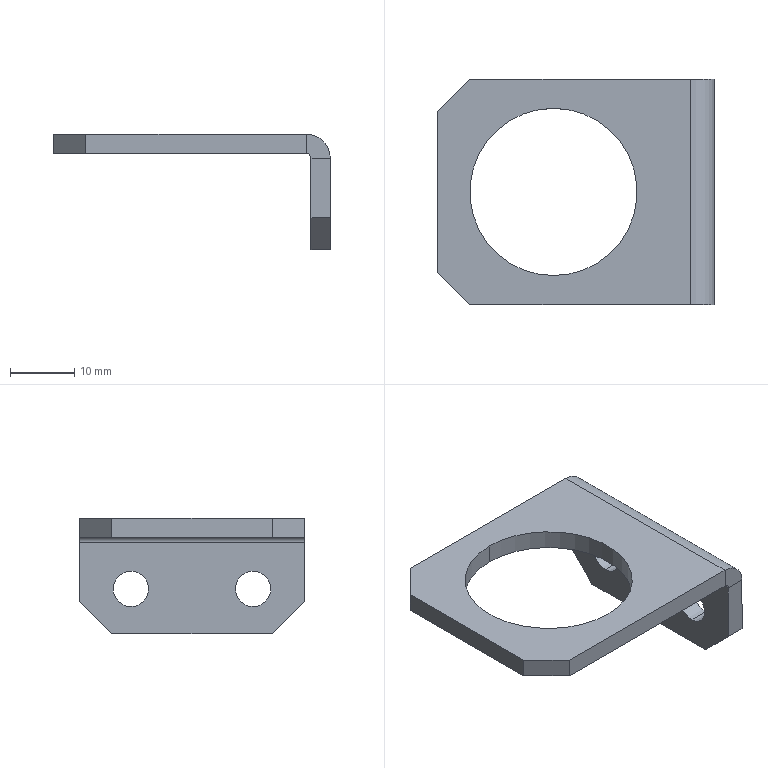Component | SolidWorks | 14-1 | 1 solid | 24 faces | box 43 x 35 x 18 mm | volume 4104 mm3 | plane 16 | cylinder 8 | commonest cylinder face diameters 5.5 x4 26 x2 1.473 x1 7.473 x1
STEP:
#1=COLOUR_RGB('',0.7922,0.8196,0.9333);
#2=FILL_AREA_STYLE_COLOUR('',#1);
#3=FILL_AREA_STYLE('',(#2));
#4=SURFACE_STYLE_FILL_AREA(#3);
#5=SURFACE_SIDE_STYLE('',(#4));
#6=SURFACE_STYLE_USAGE(.BOTH.,#5);
#7=PRESENTATION_STYLE_ASSIGNMENT((#6));
#8=CARTESIAN_POINT('',(-3.051,-1.535,8.061));
#9=VERTEX_POINT('',#8);
#10=CARTESIAN_POINT('',(-3.051,-1.535,7.844));
#11=VERTEX_POINT('',#10);
#12=CARTESIAN_POINT('',(-3.051,-1.535,7.953));
#13=DIRECTION('',(-1.,-0.,0.));
#14=DIRECTION('',(0.,0.,-1.));
#15=AXIS2_PLACEMENT_3D('',#12,#13,#14);
#16=CIRCLE('',#15,0.1083);
#17=EDGE_CURVE('',#9,#11,#16,.T.);
#18=ORIENTED_EDGE('',*,*,#17,.F.);
#19=CARTESIAN_POINT('',(-3.169,-1.535,8.061));
#20=VERTEX_POINT('',#19);
#21=CARTESIAN_POINT('',(-2.776,-1.535,8.061));
#22=DIRECTION('',(-1.,-0.,0.));
#23=VECTOR('',#22,39.37);
#24=LINE('',#21,#23);
#25=EDGE_CURVE('',#9,#20,#24,.T.);
#26=ORIENTED_EDGE('',*,*,#25,.T.);
#27=CARTESIAN_POINT('',(-3.169,-1.535,7.844));
#28=VERTEX_POINT('',#27);
#29=CARTESIAN_POINT('',(-3.169,-1.535,7.953));
#30=DIRECTION('',(-1.,-0.,0.));
#31=DIRECTION('',(0.,0.,-1.));
#32=AXIS2_PLACEMENT_3D('',#29,#30,#31);
#33=CIRCLE('',#32,0.1083);
#34=EDGE_CURVE('',#20,#28,#33,.T.);
#35=ORIENTED_EDGE('',*,*,#34,.T.);
#36=CARTESIAN_POINT('',(-2.776,-1.535,7.844));
#37=DIRECTION('',(-1.,-0.,0.));
#38=VECTOR('',#37,39.37);
#39=LINE('',#36,#38);
#40=EDGE_CURVE('',#11,#28,#39,.T.);
#41=ORIENTED_EDGE('',*,*,#40,.F.);
#42=EDGE_LOOP('',(#18,#26,#35,#41));
#43=FACE_OUTER_BOUND('',#42,.T.);
#44=CARTESIAN_POINT('',(-2.776,-1.535,7.953));
#45=DIRECTION('',(-1.,-0.,0.));
#46=DIRECTION('',(0.,0.,-1.));
#47=AXIS2_PLACEMENT_3D('',#44,#45,#46);
#48=CYLINDRICAL_SURFACE('',#47,0.1083);
#49=ADVANCED_FACE('',(#43),#48,.F.);
#50=CARTESIAN_POINT('',(-3.051,-0.7874,8.061));
#51=VERTEX_POINT('',#50);
#52=CARTESIAN_POINT('',(-3.051,-0.7874,7.844));
#53=VERTEX_POINT('',#52);
#54=CARTESIAN_POINT('',(-3.051,-0.7874,7.953));
#55=DIRECTION('',(-1.,-0.,0.));
#56=DIRECTION('',(0.,0.,-1.));
#57=AXIS2_PLACEMENT_3D('',#54,#55,#56);
#58=CIRCLE('',#57,0.1083);
#59=EDGE_CURVE('',#51,#53,#58,.T.);
#60=ORIENTED_EDGE('',*,*,#59,.F.);
#61=CARTESIAN_POINT('',(-3.169,-0.7874,8.061));
#62=VERTEX_POINT('',#61);
#63=CARTESIAN_POINT('',(-2.776,-0.7874,8.061));
#64=DIRECTION('',(-1.,-0.,0.));
#65=VECTOR('',#64,39.37);
#66=LINE('',#63,#65);
#67=EDGE_CURVE('',#51,#62,#66,.T.);
#68=ORIENTED_EDGE('',*,*,#67,.T.);
#69=CARTESIAN_POINT('',(-3.169,-0.7874,7.844));
#70=VERTEX_POINT('',#69);
#71=CARTESIAN_POINT('',(-3.169,-0.7874,7.953));
#72=DIRECTION('',(-1.,-0.,0.));
#73=DIRECTION('',(0.,0.,-1.));
#74=AXIS2_PLACEMENT_3D('',#71,#72,#73);
#75=CIRCLE('',#74,0.1083);
#76=EDGE_CURVE('',#62,#70,#75,.T.);
#77=ORIENTED_EDGE('',*,*,#76,.T.);
#78=CARTESIAN_POINT('',(-2.776,-0.7874,7.844));
#79=DIRECTION('',(-1.,-0.,0.));
#80=VECTOR('',#79,39.37);
#81=LINE('',#78,#80);
#82=EDGE_CURVE('',#53,#70,#81,.T.);
#83=ORIENTED_EDGE('',*,*,#82,.F.);
#84=EDGE_LOOP('',(#60,#68,#77,#83));
#85=FACE_OUTER_BOUND('',#84,.T.);
#86=CARTESIAN_POINT('',(-2.776,-0.7874,7.953));
#87=DIRECTION('',(-1.,-0.,0.));
#88=DIRECTION('',(0.,0.,-1.));
#89=AXIS2_PLACEMENT_3D('',#86,#87,#88);
#90=CYLINDRICAL_SURFACE('',#89,0.1083);
#91=ADVANCED_FACE('',(#85),#90,.F.);
#92=CARTESIAN_POINT('',(-4.035,-0.6496,8.386));
#93=VERTEX_POINT('',#92);
#94=CARTESIAN_POINT('',(-4.035,-1.673,8.386));
#95=VERTEX_POINT('',#94);
#96=CARTESIAN_POINT('',(-4.035,-1.161,8.386));
#97=DIRECTION('',(-0.,-0.,-1.));
#98=DIRECTION('',(0.,-1.,0.));
#99=AXIS2_PLACEMENT_3D('',#96,#97,#98);
#100=CIRCLE('',#99,0.5118);
#101=EDGE_CURVE('',#93,#95,#100,.T.);
#102=ORIENTED_EDGE('',*,*,#101,.F.);
#103=CARTESIAN_POINT('',(-4.035,-0.6496,8.268));
#104=VERTEX_POINT('',#103);
#105=CARTESIAN_POINT('',(-4.035,-0.6496,8.386));
#106=DIRECTION('',(-0.,-0.,-1.));
#107=VECTOR('',#106,39.37);
#108=LINE('',#105,#107);
#109=EDGE_CURVE('',#93,#104,#108,.T.);
#110=ORIENTED_EDGE('',*,*,#109,.T.);
#111=CARTESIAN_POINT('',(-4.035,-1.673,8.268));
#112=VERTEX_POINT('',#111);
#113=CARTESIAN_POINT('',(-4.035,-1.161,8.268));
#114=DIRECTION('',(-0.,-0.,-1.));
#115=DIRECTION('',(0.,-1.,0.));
#116=AXIS2_PLACEMENT_3D('',#113,#114,#115);
#117=CIRCLE('',#116,0.5118);
#118=EDGE_CURVE('',#104,#112,#117,.T.);
#119=ORIENTED_EDGE('',*,*,#118,.T.);
#120=CARTESIAN_POINT('',(-4.035,-1.673,8.386));
#121=DIRECTION('',(-0.,-0.,-1.));
#122=VECTOR('',#121,39.37);
#123=LINE('',#120,#122);
#124=EDGE_CURVE('',#95,#112,#123,.T.);
#125=ORIENTED_EDGE('',*,*,#124,.F.);
#126=EDGE_LOOP('',(#102,#110,#119,#125));
#127=FACE_OUTER_BOUND('',#126,.T.);
#128=CARTESIAN_POINT('',(-4.035,-1.161,8.386));
#129=DIRECTION('',(-0.,-0.,-1.));
#130=DIRECTION('',(0.,-1.,0.));
#131=AXIS2_PLACEMENT_3D('',#128,#129,#130);
#132=CYLINDRICAL_SURFACE('',#131,0.5118);
#133=ADVANCED_FACE('',(#127),#132,.F.);
#134=CARTESIAN_POINT('',(-3.198,-1.85,8.268));
#135=VERTEX_POINT('',#134);
#136=CARTESIAN_POINT('',(-3.198,-1.85,8.386));
#137=VERTEX_POINT('',#136);
#138=CARTESIAN_POINT('',(-3.198,-1.85,8.268));
#139=DIRECTION('',(0.,0.,1.));
#140=VECTOR('',#139,39.37);
#141=LINE('',#138,#140);
#142=EDGE_CURVE('',#135,#137,#141,.T.);
#143=ORIENTED_EDGE('',*,*,#142,.F.);
#144=CARTESIAN_POINT('',(-3.169,-1.85,8.239));
#145=VERTEX_POINT('',#144);
#146=CARTESIAN_POINT('',(-3.198,-1.85,8.239));
#147=DIRECTION('',(0.,-1.,0.));
#148=DIRECTION('',(0.,0.,-1.));
#149=AXIS2_PLACEMENT_3D('',#146,#147,#148);
#150=CIRCLE('',#149,0.029);
#151=EDGE_CURVE('',#145,#135,#150,.T.);
#152=ORIENTED_EDGE('',*,*,#151,.F.);
#153=CARTESIAN_POINT('',(-3.051,-1.85,8.239));
#154=VERTEX_POINT('',#153);
#155=CARTESIAN_POINT('',(-3.051,-1.85,8.239));
#156=DIRECTION('',(-1.,-0.,0.));
#157=VECTOR('',#156,39.37);
#158=LINE('',#155,#157);
#159=EDGE_CURVE('',#154,#145,#158,.T.);
#160=ORIENTED_EDGE('',*,*,#159,.F.);
#161=CARTESIAN_POINT('',(-3.198,-1.85,8.239));
#162=DIRECTION('',(0.,-1.,0.));
#163=DIRECTION('',(0.,0.,1.));
#164=AXIS2_PLACEMENT_3D('',#161,#162,#163);
#165=CIRCLE('',#164,0.1471);
#166=EDGE_CURVE('',#154,#137,#165,.T.);
#167=ORIENTED_EDGE('',*,*,#166,.T.);
#168=EDGE_LOOP('',(#143,#152,#160,#167));
#169=FACE_OUTER_BOUND('',#168,.T.);
#170=CARTESIAN_POINT('',(-3.198,-1.85,8.268));
#171=DIRECTION('',(0.,-1.,0.));
#172=DIRECTION('',(0.,0.,1.));
#173=AXIS2_PLACEMENT_3D('',#170,#171,#172);
#174=PLANE('',#173);
#175=ADVANCED_FACE('',(#169),#174,.T.);
#176=CARTESIAN_POINT('',(-4.547,-1.85,8.386));
#177=VERTEX_POINT('',#176);
#178=CARTESIAN_POINT('',(-3.169,-1.85,8.386));
#179=DIRECTION('',(-1.,-0.,0.));
#180=VECTOR('',#179,39.37);
#181=LINE('',#178,#180);
#182=EDGE_CURVE('',#137,#177,#181,.T.);
#183=ORIENTED_EDGE('',*,*,#182,.T.);
#184=CARTESIAN_POINT('',(-4.547,-1.85,8.268));
#185=VERTEX_POINT('',#184);
#186=CARTESIAN_POINT('',(-4.547,-1.85,8.239));
#187=DIRECTION('',(-0.,-0.,-1.));
#188=VECTOR('',#187,39.37);
#189=LINE('',#186,#188);
#190=EDGE_CURVE('',#177,#185,#189,.T.);
#191=ORIENTED_EDGE('',*,*,#190,.T.);
#192=CARTESIAN_POINT('',(-3.169,-1.85,8.268));
#193=DIRECTION('',(-1.,-0.,0.));
#194=VECTOR('',#193,39.37);
#195=LINE('',#192,#194);
#196=EDGE_CURVE('',#135,#185,#195,.T.);
#197=ORIENTED_EDGE('',*,*,#196,.F.);
#198=ORIENTED_EDGE('',*,*,#142,.T.);
#199=EDGE_LOOP('',(#183,#191,#197,#198));
#200=FACE_OUTER_BOUND('',#199,.T.);
#201=CARTESIAN_POINT('',(-3.051,-1.85,8.239));
#202=DIRECTION('',(0.,-1.,0.));
#203=DIRECTION('',(0.,0.,1.));
#204=AXIS2_PLACEMENT_3D('',#201,#202,#203);
#205=PLANE('',#204);
#206=ADVANCED_FACE('',(#200),#205,.T.);
#207=CARTESIAN_POINT('',(-3.169,-0.4724,8.239));
#208=VERTEX_POINT('',#207);
#209=CARTESIAN_POINT('',(-3.051,-0.4724,8.239));
#210=VERTEX_POINT('',#209);
#211=CARTESIAN_POINT('',(-3.169,-0.4724,8.239));
#212=DIRECTION('',(1.,0.,-0.));
#213=VECTOR('',#212,39.37);
#214=LINE('',#211,#213);
#215=EDGE_CURVE('',#208,#210,#214,.T.);
#216=ORIENTED_EDGE('',*,*,#215,.F.);
#217=CARTESIAN_POINT('',(-3.198,-0.4724,8.268));
#218=VERTEX_POINT('',#217);
#219=CARTESIAN_POINT('',(-3.198,-0.4724,8.239));
#220=DIRECTION('',(0.,-1.,0.));
#221=DIRECTION('',(0.,0.,-1.));
#222=AXIS2_PLACEMENT_3D('',#219,#220,#221);
#223=CIRCLE('',#222,0.029);
#224=EDGE_CURVE('',#208,#218,#223,.T.);
#225=ORIENTED_EDGE('',*,*,#224,.T.);
#226=CARTESIAN_POINT('',(-3.198,-0.4724,8.386));
#227=VERTEX_POINT('',#226);
#228=CARTESIAN_POINT('',(-3.198,-0.4724,8.386));
#229=DIRECTION('',(-0.,-0.,-1.));
#230=VECTOR('',#229,39.37);
#231=LINE('',#228,#230);
#232=EDGE_CURVE('',#227,#218,#231,.T.);
#233=ORIENTED_EDGE('',*,*,#232,.F.);
#234=CARTESIAN_POINT('',(-3.198,-0.4724,8.239));
#235=DIRECTION('',(0.,-1.,0.));
#236=DIRECTION('',(0.,0.,1.));
#237=AXIS2_PLACEMENT_3D('',#234,#235,#236);
#238=CIRCLE('',#237,0.1471);
#239=EDGE_CURVE('',#210,#227,#238,.T.);
#240=ORIENTED_EDGE('',*,*,#239,.F.);
#241=EDGE_LOOP('',(#216,#225,#233,#240));
#242=FACE_OUTER_BOUND('',#241,.T.);
#243=CARTESIAN_POINT('',(-3.169,-0.4724,8.239));
#244=DIRECTION('',(-0.,1.,-0.));
#245=DIRECTION('',(-0.,-0.,-1.));
#246=AXIS2_PLACEMENT_3D('',#243,#244,#245);
#247=PLANE('',#246);
#248=ADVANCED_FACE('',(#242),#247,.T.);
#249=CARTESIAN_POINT('',(-3.051,-0.4724,7.874));
#250=VERTEX_POINT('',#249);
#251=CARTESIAN_POINT('',(-3.051,-0.4724,7.677));
#252=DIRECTION('',(0.,0.,1.));
#253=VECTOR('',#252,39.37);
#254=LINE('',#251,#253);
#255=EDGE_CURVE('',#250,#210,#254,.T.);
#256=ORIENTED_EDGE('',*,*,#255,.F.);
#257=CARTESIAN_POINT('',(-3.169,-0.4724,7.874));
#258=VERTEX_POINT('',#257);
#259=CARTESIAN_POINT('',(-3.198,-0.4724,7.874));
#260=DIRECTION('',(-1.,-0.,0.));
#261=VECTOR('',#260,39.37);
#262=LINE('',#259,#261);
#263=EDGE_CURVE('',#250,#258,#262,.T.);
#264=ORIENTED_EDGE('',*,*,#263,.T.);
#265=CARTESIAN_POINT('',(-3.169,-0.4724,7.677));
#266=DIRECTION('',(0.,0.,1.));
#267=VECTOR('',#266,39.37);
#268=LINE('',#265,#267);
#269=EDGE_CURVE('',#258,#208,#268,.T.);
#270=ORIENTED_EDGE('',*,*,#269,.T.);
#271=ORIENTED_EDGE('',*,*,#215,.T.);
#272=EDGE_LOOP('',(#256,#264,#270,#271));
#273=FACE_OUTER_BOUND('',#272,.T.);
#274=CARTESIAN_POINT('',(-3.198,-0.4724,8.386));
#275=DIRECTION('',(-0.,1.,-0.));
#276=DIRECTION('',(-0.,-0.,-1.));
#277=AXIS2_PLACEMENT_3D('',#274,#275,#276);
#278=PLANE('',#277);
#279=ADVANCED_FACE('',(#273),#278,.T.);
#280=CARTESIAN_POINT('',(-4.035,-1.161,8.386));
#281=DIRECTION('',(-0.,-0.,-1.));
#282=DIRECTION('',(0.,-1.,0.));
#283=AXIS2_PLACEMENT_3D('',#280,#281,#282);
#284=CIRCLE('',#283,0.5118);
#285=EDGE_CURVE('',#95,#93,#284,.T.);
#286=ORIENTED_EDGE('',*,*,#285,.T.);
#287=ORIENTED_EDGE('',*,*,#101,.T.);
#288=EDGE_LOOP('',(#286,#287));
#289=FACE_BOUND('',#288,.T.);
#290=CARTESIAN_POINT('',(-4.547,-0.4724,8.386));
#291=VERTEX_POINT('',#290);
#292=CARTESIAN_POINT('',(-3.169,-0.4724,8.386));
#293=DIRECTION('',(-1.,-0.,0.));
#294=VECTOR('',#293,39.37);
#295=LINE('',#292,#294);
#296=EDGE_CURVE('',#227,#291,#295,.T.);
#297=ORIENTED_EDGE('',*,*,#296,.T.);
#298=CARTESIAN_POINT('',(-4.744,-0.6693,8.386));
#299=VERTEX_POINT('',#298);
#300=CARTESIAN_POINT('',(-4.547,-0.4724,8.386));
#301=DIRECTION('',(-0.7071,-0.7071,0.));
#302=VECTOR('',#301,39.37);
#303=LINE('',#300,#302);
#304=EDGE_CURVE('',#291,#299,#303,.T.);
#305=ORIENTED_EDGE('',*,*,#304,.T.);
#306=CARTESIAN_POINT('',(-4.744,-1.654,8.386));
#307=VERTEX_POINT('',#306);
#308=CARTESIAN_POINT('',(-4.744,-1.85,8.386));
#309=DIRECTION('',(-0.,1.,-0.));
#310=VECTOR('',#309,39.37);
#311=LINE('',#308,#310);
#312=EDGE_CURVE('',#307,#299,#311,.T.);
#313=ORIENTED_EDGE('',*,*,#312,.F.);
#314=CARTESIAN_POINT('',(-4.744,-1.654,8.386));
#315=DIRECTION('',(0.7071,-0.7071,0.));
#316=VECTOR('',#315,39.37);
#317=LINE('',#314,#316);
#318=EDGE_CURVE('',#307,#177,#317,.T.);
#319=ORIENTED_EDGE('',*,*,#318,.T.);
#320=ORIENTED_EDGE('',*,*,#182,.F.);
#321=CARTESIAN_POINT('',(-3.198,-1.85,8.386));
#322=DIRECTION('',(-0.,1.,-0.));
#323=VECTOR('',#322,39.37);
#324=LINE('',#321,#323);
#325=EDGE_CURVE('',#137,#227,#324,.T.);
#326=ORIENTED_EDGE('',*,*,#325,.T.);
#327=EDGE_LOOP('',(#297,#305,#313,#319,#320,#326));
#328=FACE_OUTER_BOUND('',#327,.T.);
#329=CARTESIAN_POINT('',(-3.169,-1.85,8.386));
#330=DIRECTION('',(-0.,-0.,-1.));
#331=DIRECTION('',(0.,-1.,0.));
#332=AXIS2_PLACEMENT_3D('',#329,#330,#331);
#333=PLANE('',#332);
#334=ADVANCED_FACE('',(#289,#328),#333,.F.);
#335=ORIENTED_EDGE('',*,*,#312,.T.);
#336=CARTESIAN_POINT('',(-4.744,-0.6693,8.268));
#337=VERTEX_POINT('',#336);
#338=CARTESIAN_POINT('',(-4.744,-0.6693,8.268));
#339=DIRECTION('',(-0.,-0.,-1.));
#340=VECTOR('',#339,39.37);
#341=LINE('',#338,#340);
#342=EDGE_CURVE('',#299,#337,#341,.T.);
#343=ORIENTED_EDGE('',*,*,#342,.T.);
#344=CARTESIAN_POINT('',(-4.744,-1.654,8.268));
#345=VERTEX_POINT('',#344);
#346=CARTESIAN_POINT('',(-4.744,-1.85,8.268));
#347=DIRECTION('',(-0.,1.,-0.));
#348=VECTOR('',#347,39.37);
#349=LINE('',#346,#348);
#350=EDGE_CURVE('',#345,#337,#349,.T.);
#351=ORIENTED_EDGE('',*,*,#350,.F.);
#352=CARTESIAN_POINT('',(-4.744,-1.654,8.268));
#353=DIRECTION('',(0.,0.,1.));
#354=VECTOR('',#353,39.37);
#355=LINE('',#352,#354);
#356=EDGE_CURVE('',#345,#307,#355,.T.);
#357=ORIENTED_EDGE('',*,*,#356,.T.);
#358=EDGE_LOOP('',(#335,#343,#351,#357));
#359=FACE_OUTER_BOUND('',#358,.T.);
#360=CARTESIAN_POINT('',(-4.744,-1.85,8.268));
#361=DIRECTION('',(-1.,-0.,0.));
#362=DIRECTION('',(-0.,-0.,-1.));
#363=AXIS2_PLACEMENT_3D('',#360,#361,#362);
#364=PLANE('',#363);
#365=ADVANCED_FACE('',(#359),#364,.T.);
#366=CARTESIAN_POINT('',(-4.035,-1.161,8.268));
#367=DIRECTION('',(-0.,-0.,-1.));
#368=DIRECTION('',(0.,-1.,0.));
#369=AXIS2_PLACEMENT_3D('',#366,#367,#368);
#370=CIRCLE('',#369,0.5118);
#371=EDGE_CURVE('',#112,#104,#370,.T.);
#372=ORIENTED_EDGE('',*,*,#371,.F.);
#373=ORIENTED_EDGE('',*,*,#118,.F.);
#374=EDGE_LOOP('',(#372,#373));
#375=FACE_BOUND('',#374,.T.);
#376=ORIENTED_EDGE('',*,*,#350,.T.);
#377=CARTESIAN_POINT('',(-4.547,-0.4724,8.268));
#378=VERTEX_POINT('',#377);
#379=CARTESIAN_POINT('',(-4.547,-0.4724,8.268));
#380=DIRECTION('',(0.7071,0.7071,-0.));
#381=VECTOR('',#380,39.37);
#382=LINE('',#379,#381);
#383=EDGE_CURVE('',#337,#378,#382,.T.);
#384=ORIENTED_EDGE('',*,*,#383,.T.);
#385=CARTESIAN_POINT('',(-3.169,-0.4724,8.268));
#386=DIRECTION('',(-1.,-0.,0.));
#387=VECTOR('',#386,39.37);
#388=LINE('',#385,#387);
#389=EDGE_CURVE('',#218,#378,#388,.T.);
#390=ORIENTED_EDGE('',*,*,#389,.F.);
#391=CARTESIAN_POINT('',(-3.198,-1.85,8.268));
#392=DIRECTION('',(-0.,1.,-0.));
#393=VECTOR('',#392,39.37);
#394=LINE('',#391,#393);
#395=EDGE_CURVE('',#135,#218,#394,.T.);
#396=ORIENTED_EDGE('',*,*,#395,.F.);
#397=ORIENTED_EDGE('',*,*,#196,.T.);
#398=CARTESIAN_POINT('',(-3.858,-2.539,8.268));
#399=DIRECTION('',(-0.7071,0.7071,-0.));
#400=VECTOR('',#399,39.37);
#401=LINE('',#398,#400);
#402=EDGE_CURVE('',#185,#345,#401,.T.);
#403=ORIENTED_EDGE('',*,*,#402,.T.);
#404=EDGE_LOOP('',(#376,#384,#390,#396,#397,#403));
#405=FACE_OUTER_BOUND('',#404,.T.);
#406=CARTESIAN_POINT('',(-3.169,-1.85,8.268));
#407=DIRECTION('',(-0.,-0.,-1.));
#408=DIRECTION('',(0.,-1.,0.));
#409=AXIS2_PLACEMENT_3D('',#406,#407,#408);
#410=PLANE('',#409);
#411=ADVANCED_FACE('',(#375,#405),#410,.T.);
#412=ORIENTED_EDGE('',*,*,#224,.F.);
#413=CARTESIAN_POINT('',(-3.169,-1.85,8.239));
#414=DIRECTION('',(-0.,1.,-0.));
#415=VECTOR('',#414,39.37);
#416=LINE('',#413,#415);
#417=EDGE_CURVE('',#145,#208,#416,.T.);
#418=ORIENTED_EDGE('',*,*,#417,.F.);
#419=ORIENTED_EDGE('',*,*,#151,.T.);
#420=ORIENTED_EDGE('',*,*,#395,.T.);
#421=EDGE_LOOP('',(#412,#418,#419,#420));
#422=FACE_OUTER_BOUND('',#421,.T.);
#423=CARTESIAN_POINT('',(-3.198,-1.85,8.239));
#424=DIRECTION('',(-0.,1.,-0.));
#425=DIRECTION('',(0.,0.,-1.));
#426=AXIS2_PLACEMENT_3D('',#423,#424,#425);
#427=CYLINDRICAL_SURFACE('',#426,0.029);
#428=ADVANCED_FACE('',(#422),#427,.F.);
#429=CARTESIAN_POINT('',(-3.169,-1.535,7.953));
#430=DIRECTION('',(-1.,-0.,0.));
#431=DIRECTION('',(0.,0.,-1.));
#432=AXIS2_PLACEMENT_3D('',#429,#430,#431);
#433=CIRCLE('',#432,0.1083);
#434=EDGE_CURVE('',#28,#20,#433,.T.);
#435=ORIENTED_EDGE('',*,*,#434,.F.);
#436=ORIENTED_EDGE('',*,*,#34,.F.);
#437=EDGE_LOOP('',(#435,#436));
#438=FACE_BOUND('',#437,.T.);
#439=CARTESIAN_POINT('',(-3.169,-0.7874,7.953));
#440=DIRECTION('',(-1.,-0.,0.));
#441=DIRECTION('',(0.,0.,-1.));
#442=AXIS2_PLACEMENT_3D('',#439,#440,#441);
#443=CIRCLE('',#442,0.1083);
#444=EDGE_CURVE('',#70,#62,#443,.T.);
#445=ORIENTED_EDGE('',*,*,#444,.F.);
#446=ORIENTED_EDGE('',*,*,#76,.F.);
#447=EDGE_LOOP('',(#445,#446));
#448=FACE_BOUND('',#447,.T.);
#449=ORIENTED_EDGE('',*,*,#269,.F.);
#450=CARTESIAN_POINT('',(-3.169,-0.6693,7.677));
#451=VERTEX_POINT('',#450);
#452=CARTESIAN_POINT('',(-3.169,-1.26,7.087));
#453=DIRECTION('',(-0.,-0.7071,-0.7071));
#454=VECTOR('',#453,39.37);
#455=LINE('',#452,#454);
#456=EDGE_CURVE('',#258,#451,#455,.T.);
#457=ORIENTED_EDGE('',*,*,#456,.T.);
#458=CARTESIAN_POINT('',(-3.169,-1.654,7.677));
#459=VERTEX_POINT('',#458);
#460=CARTESIAN_POINT('',(-3.169,-1.85,7.677));
#461=DIRECTION('',(-0.,1.,-0.));
#462=VECTOR('',#461,39.37);
#463=LINE('',#460,#462);
#464=EDGE_CURVE('',#459,#451,#463,.T.);
#465=ORIENTED_EDGE('',*,*,#464,.F.);
#466=CARTESIAN_POINT('',(-3.169,-1.85,7.874));
#467=VERTEX_POINT('',#466);
#468=CARTESIAN_POINT('',(-3.169,-1.752,7.776));
#469=DIRECTION('',(0.,-0.7071,0.7071));
#470=VECTOR('',#469,39.37);
#471=LINE('',#468,#470);
#472=EDGE_CURVE('',#459,#467,#471,.T.);
#473=ORIENTED_EDGE('',*,*,#472,.T.);
#474=CARTESIAN_POINT('',(-3.169,-1.85,7.677));
#475=DIRECTION('',(0.,0.,1.));
#476=VECTOR('',#475,39.37);
#477=LINE('',#474,#476);
#478=EDGE_CURVE('',#467,#145,#477,.T.);
#479=ORIENTED_EDGE('',*,*,#478,.T.);
#480=ORIENTED_EDGE('',*,*,#417,.T.);
#481=EDGE_LOOP('',(#449,#457,#465,#473,#479,#480));
#482=FACE_OUTER_BOUND('',#481,.T.);
#483=CARTESIAN_POINT('',(-3.169,-1.85,7.677));
#484=DIRECTION('',(-1.,-0.,0.));
#485=DIRECTION('',(-0.,-0.,-1.));
#486=AXIS2_PLACEMENT_3D('',#483,#484,#485);
#487=PLANE('',#486);
#488=ADVANCED_FACE('',(#438,#448,#482),#487,.T.);
#489=ORIENTED_EDGE('',*,*,#464,.T.);
#490=CARTESIAN_POINT('',(-3.051,-0.6693,7.677));
#491=VERTEX_POINT('',#490);
#492=CARTESIAN_POINT('',(-3.051,-0.6693,7.677));
#493=DIRECTION('',(1.,0.,-0.));
#494=VECTOR('',#493,39.37);
#495=LINE('',#492,#494);
#496=EDGE_CURVE('',#451,#491,#495,.T.);
#497=ORIENTED_EDGE('',*,*,#496,.T.);
#498=CARTESIAN_POINT('',(-3.051,-1.654,7.677));
#499=VERTEX_POINT('',#498);
#500=CARTESIAN_POINT('',(-3.051,-1.85,7.677));
#501=DIRECTION('',(-0.,1.,-0.));
#502=VECTOR('',#501,39.37);
#503=LINE('',#500,#502);
#504=EDGE_CURVE('',#499,#491,#503,.T.);
#505=ORIENTED_EDGE('',*,*,#504,.F.);
#506=CARTESIAN_POINT('',(-3.169,-1.654,7.677));
#507=DIRECTION('',(-1.,-0.,0.));
#508=VECTOR('',#507,39.37);
#509=LINE('',#506,#508);
#510=EDGE_CURVE('',#499,#459,#509,.T.);
#511=ORIENTED_EDGE('',*,*,#510,.T.);
#512=EDGE_LOOP('',(#489,#497,#505,#511));
#513=FACE_OUTER_BOUND('',#512,.T.);
#514=CARTESIAN_POINT('',(-3.051,-1.85,7.677));
#515=DIRECTION('',(-0.,-0.,-1.));
#516=DIRECTION('',(0.,-1.,0.));
#517=AXIS2_PLACEMENT_3D('',#514,#515,#516);
#518=PLANE('',#517);
#519=ADVANCED_FACE('',(#513),#518,.T.);
#520=CARTESIAN_POINT('',(-3.051,-1.535,7.953));
#521=DIRECTION('',(-1.,-0.,0.));
#522=DIRECTION('',(0.,0.,-1.));
#523=AXIS2_PLACEMENT_3D('',#520,#521,#522);
#524=CIRCLE('',#523,0.1083);
#525=EDGE_CURVE('',#11,#9,#524,.T.);
#526=ORIENTED_EDGE('',*,*,#525,.T.);
#527=ORIENTED_EDGE('',*,*,#17,.T.);
#528=EDGE_LOOP('',(#526,#527));
#529=FACE_BOUND('',#528,.T.);
#530=CARTESIAN_POINT('',(-3.051,-0.7874,7.953));
#531=DIRECTION('',(-1.,-0.,0.));
#532=DIRECTION('',(0.,0.,-1.));
#533=AXIS2_PLACEMENT_3D('',#530,#531,#532);
#534=CIRCLE('',#533,0.1083);
#535=EDGE_CURVE('',#53,#51,#534,.T.);
#536=ORIENTED_EDGE('',*,*,#535,.T.);
#537=ORIENTED_EDGE('',*,*,#59,.T.);
#538=EDGE_LOOP('',(#536,#537));
#539=FACE_BOUND('',#538,.T.);
#540=ORIENTED_EDGE('',*,*,#504,.T.);
#541=CARTESIAN_POINT('',(-3.051,-0.4724,7.874));
#542=DIRECTION('',(0.,0.7071,0.7071));
#543=VECTOR('',#542,39.37);
#544=LINE('',#541,#543);
#545=EDGE_CURVE('',#491,#250,#544,.T.);
#546=ORIENTED_EDGE('',*,*,#545,.T.);
#547=ORIENTED_EDGE('',*,*,#255,.T.);
#548=CARTESIAN_POINT('',(-3.051,-1.85,8.239));
#549=DIRECTION('',(-0.,1.,-0.));
#550=VECTOR('',#549,39.37);
#551=LINE('',#548,#550);
#552=EDGE_CURVE('',#154,#210,#551,.T.);
#553=ORIENTED_EDGE('',*,*,#552,.F.);
#554=CARTESIAN_POINT('',(-3.051,-1.85,7.874));
#555=VERTEX_POINT('',#554);
#556=CARTESIAN_POINT('',(-3.051,-1.85,7.677));
#557=DIRECTION('',(0.,0.,1.));
#558=VECTOR('',#557,39.37);
#559=LINE('',#556,#558);
#560=EDGE_CURVE('',#555,#154,#559,.T.);
#561=ORIENTED_EDGE('',*,*,#560,.F.);
#562=CARTESIAN_POINT('',(-3.051,-1.654,7.677));
#563=DIRECTION('',(-0.,0.7071,-0.7071));
#564=VECTOR('',#563,39.37);
#565=LINE('',#562,#564);
#566=EDGE_CURVE('',#555,#499,#565,.T.);
#567=ORIENTED_EDGE('',*,*,#566,.T.);
#568=EDGE_LOOP('',(#540,#546,#547,#553,#561,#567));
#569=FACE_OUTER_BOUND('',#568,.T.);
#570=CARTESIAN_POINT('',(-3.051,-1.85,7.677));
#571=DIRECTION('',(-1.,-0.,0.));
#572=DIRECTION('',(-0.,-0.,-1.));
#573=AXIS2_PLACEMENT_3D('',#570,#571,#572);
#574=PLANE('',#573);
#575=ADVANCED_FACE('',(#529,#539,#569),#574,.F.);
#576=ORIENTED_EDGE('',*,*,#239,.T.);
#577=ORIENTED_EDGE('',*,*,#325,.F.);
#578=ORIENTED_EDGE('',*,*,#166,.F.);
#579=ORIENTED_EDGE('',*,*,#552,.T.);
#580=EDGE_LOOP('',(#576,#577,#578,#579));
#581=FACE_OUTER_BOUND('',#580,.T.);
#582=CARTESIAN_POINT('',(-3.198,-1.85,8.239));
#583=DIRECTION('',(-0.,1.,-0.));
#584=DIRECTION('',(0.,0.,-1.));
#585=AXIS2_PLACEMENT_3D('',#582,#583,#584);
#586=CYLINDRICAL_SURFACE('',#585,0.1471);
#587=ADVANCED_FACE('',(#581),#586,.T.);
#588=ORIENTED_EDGE('',*,*,#478,.F.);
#589=CARTESIAN_POINT('',(-3.051,-1.85,7.874));
#590=DIRECTION('',(1.,0.,-0.));
#591=VECTOR('',#590,39.37);
#592=LINE('',#589,#591);
#593=EDGE_CURVE('',#467,#555,#592,.T.);
#594=ORIENTED_EDGE('',*,*,#593,.T.);
#595=ORIENTED_EDGE('',*,*,#560,.T.);
#596=ORIENTED_EDGE('',*,*,#159,.T.);
#597=EDGE_LOOP('',(#588,#594,#595,#596));
#598=FACE_OUTER_BOUND('',#597,.T.);
#599=CARTESIAN_POINT('',(-3.198,-1.85,8.239));
#600=DIRECTION('',(-0.,1.,-0.));
#601=DIRECTION('',(-0.,-0.,-1.));
#602=AXIS2_PLACEMENT_3D('',#599,#600,#601);
#603=PLANE('',#602);
#604=ADVANCED_FACE('',(#598),#603,.F.);
#605=ORIENTED_EDGE('',*,*,#389,.T.);
#606=CARTESIAN_POINT('',(-4.547,-0.4724,8.239));
#607=DIRECTION('',(0.,0.,1.));
#608=VECTOR('',#607,39.37);
#609=LINE('',#606,#608);
#610=EDGE_CURVE('',#378,#291,#609,.T.);
#611=ORIENTED_EDGE('',*,*,#610,.T.);
#612=ORIENTED_EDGE('',*,*,#296,.F.);
#613=ORIENTED_EDGE('',*,*,#232,.T.);
#614=EDGE_LOOP('',(#605,#611,#612,#613));
#615=FACE_OUTER_BOUND('',#614,.T.);
#616=CARTESIAN_POINT('',(-3.198,-0.4724,8.239));
#617=DIRECTION('',(-0.,1.,-0.));
#618=DIRECTION('',(-0.,-0.,-1.));
#619=AXIS2_PLACEMENT_3D('',#616,#617,#618);
#620=PLANE('',#619);
#621=ADVANCED_FACE('',(#615),#620,.T.);
#622=ORIENTED_EDGE('',*,*,#109,.F.);
#623=ORIENTED_EDGE('',*,*,#285,.F.);
#624=ORIENTED_EDGE('',*,*,#124,.T.);
#625=ORIENTED_EDGE('',*,*,#371,.T.);
#626=EDGE_LOOP('',(#622,#623,#624,#625));
#627=FACE_OUTER_BOUND('',#626,.T.);
#628=CARTESIAN_POINT('',(-4.035,-1.161,8.386));
#629=DIRECTION('',(-0.,-0.,-1.));
#630=DIRECTION('',(0.,-1.,0.));
#631=AXIS2_PLACEMENT_3D('',#628,#629,#630);
#632=CYLINDRICAL_SURFACE('',#631,0.5118);
#633=ADVANCED_FACE('',(#627),#632,.F.);
#634=ORIENTED_EDGE('',*,*,#383,.F.);
#635=ORIENTED_EDGE('',*,*,#342,.F.);
#636=ORIENTED_EDGE('',*,*,#304,.F.);
#637=ORIENTED_EDGE('',*,*,#610,.F.);
#638=EDGE_LOOP('',(#634,#635,#636,#637));
#639=FACE_OUTER_BOUND('',#638,.T.);
#640=CARTESIAN_POINT('',(-4.547,-0.4724,8.239));
#641=DIRECTION('',(0.7071,-0.7071,0.));
#642=DIRECTION('',(0.,0.,1.));
#643=AXIS2_PLACEMENT_3D('',#640,#641,#642);
#644=PLANE('',#643);
#645=ADVANCED_FACE('',(#639),#644,.F.);
#646=ORIENTED_EDGE('',*,*,#402,.F.);
#647=ORIENTED_EDGE('',*,*,#190,.F.);
#648=ORIENTED_EDGE('',*,*,#318,.F.);
#649=ORIENTED_EDGE('',*,*,#356,.F.);
#650=EDGE_LOOP('',(#646,#647,#648,#649));
#651=FACE_OUTER_BOUND('',#650,.T.);
#652=CARTESIAN_POINT('',(-4.744,-1.654,8.268));
#653=DIRECTION('',(0.7071,0.7071,-0.));
#654=DIRECTION('',(0.,0.,1.));
#655=AXIS2_PLACEMENT_3D('',#652,#653,#654);
#656=PLANE('',#655);
#657=ADVANCED_FACE('',(#651),#656,.F.);
#658=ORIENTED_EDGE('',*,*,#545,.F.);
#659=ORIENTED_EDGE('',*,*,#496,.F.);
#660=ORIENTED_EDGE('',*,*,#456,.F.);
#661=ORIENTED_EDGE('',*,*,#263,.F.);
#662=EDGE_LOOP('',(#658,#659,#660,#661));
#663=FACE_OUTER_BOUND('',#662,.T.);
#664=CARTESIAN_POINT('',(-3.198,-0.4724,7.874));
#665=DIRECTION('',(0.,-0.7071,0.7071));
#666=DIRECTION('',(-1.,-0.,0.));
#667=AXIS2_PLACEMENT_3D('',#664,#665,#666);
#668=PLANE('',#667);
#669=ADVANCED_FACE('',(#663),#668,.F.);
#670=ORIENTED_EDGE('',*,*,#566,.F.);
#671=ORIENTED_EDGE('',*,*,#593,.F.);
#672=ORIENTED_EDGE('',*,*,#472,.F.);
#673=ORIENTED_EDGE('',*,*,#510,.F.);
#674=EDGE_LOOP('',(#670,#671,#672,#673));
#675=FACE_OUTER_BOUND('',#674,.T.);
#676=CARTESIAN_POINT('',(-3.051,-1.654,7.677));
#677=DIRECTION('',(-0.,-0.7071,-0.7071));
#678=DIRECTION('',(1.,0.,-0.));
#679=AXIS2_PLACEMENT_3D('',#676,#677,#678);
#680=PLANE('',#679);
#681=ADVANCED_FACE('',(#675),#680,.T.);
#682=ORIENTED_EDGE('',*,*,#67,.F.);
#683=ORIENTED_EDGE('',*,*,#535,.F.);
#684=ORIENTED_EDGE('',*,*,#82,.T.);
#685=ORIENTED_EDGE('',*,*,#444,.T.);
#686=EDGE_LOOP('',(#682,#683,#684,#685));
#687=FACE_OUTER_BOUND('',#686,.T.);
#688=CARTESIAN_POINT('',(-2.776,-0.7874,7.953));
#689=DIRECTION('',(-1.,-0.,0.));
#690=DIRECTION('',(0.,0.,-1.));
#691=AXIS2_PLACEMENT_3D('',#688,#689,#690);
#692=CYLINDRICAL_SURFACE('',#691,0.1083);
#693=ADVANCED_FACE('',(#687),#692,.F.);
#694=ORIENTED_EDGE('',*,*,#25,.F.);
#695=ORIENTED_EDGE('',*,*,#525,.F.);
#696=ORIENTED_EDGE('',*,*,#40,.T.);
#697=ORIENTED_EDGE('',*,*,#434,.T.);
#698=EDGE_LOOP('',(#694,#695,#696,#697));
#699=FACE_OUTER_BOUND('',#698,.T.);
#700=CARTESIAN_POINT('',(-2.776,-1.535,7.953));
#701=DIRECTION('',(-1.,-0.,0.));
#702=DIRECTION('',(0.,0.,-1.));
#703=AXIS2_PLACEMENT_3D('',#700,#701,#702);
#704=CYLINDRICAL_SURFACE('',#703,0.1083);
#705=ADVANCED_FACE('',(#699),#704,.F.);
#706=CLOSED_SHELL('',(#49,#91,#133,#175,#206,#248,#279,#334,#365,#411,#428,#488,#519,#575,#587,#604,#621,#633,#645,#657,#669,#681,#693,#705));
#707=MANIFOLD_SOLID_BREP('',#706);
#708=STYLED_ITEM('',(#7),#707);
#709=PRESENTATION_LAYER_ASSIGNMENT('','',(#708));
#710=CARTESIAN_POINT('',(0.,0.,0.));
#711=DIRECTION('',(0.,0.,1.));
#712=DIRECTION('',(1.,0.,0.));
#713=AXIS2_PLACEMENT_3D('',#710,#711,#712);
#714=(LENGTH_UNIT()NAMED_UNIT(*)SI_UNIT($,.METRE.));
#715=LENGTH_MEASURE_WITH_UNIT(LENGTH_MEASURE(0.0254),#714);
#716=DIMENSIONAL_EXPONENTS(1.,0.,0.,0.,0.,0.,0.);
#717=(CONVERSION_BASED_UNIT('',#715)LENGTH_UNIT()NAMED_UNIT(#716));
#718=UNCERTAINTY_MEASURE_WITH_UNIT(LENGTH_MEASURE(0.00001),#717,'','');
#719=(NAMED_UNIT(*)PLANE_ANGLE_UNIT()SI_UNIT($,.RADIAN.));
#720=(NAMED_UNIT(*)SI_UNIT($,.STERADIAN.)SOLID_ANGLE_UNIT());
#721=(GEOMETRIC_REPRESENTATION_CONTEXT(3)GLOBAL_UNCERTAINTY_ASSIGNED_CONTEXT((#718))GLOBAL_UNIT_ASSIGNED_CONTEXT((#717,#719,#720))REPRESENTATION_CONTEXT('',''));
#722=ADVANCED_BREP_SHAPE_REPRESENTATION('',(#707,#713),#721);
#723=(LENGTH_UNIT()NAMED_UNIT(*)SI_UNIT($,.METRE.));
#724=LENGTH_MEASURE_WITH_UNIT(LENGTH_MEASURE(0.0254),#723);
#725=DIMENSIONAL_EXPONENTS(1.,0.,0.,0.,0.,0.,0.);
#726=(CONVERSION_BASED_UNIT('',#724)LENGTH_UNIT()NAMED_UNIT(#725));
#727=UNCERTAINTY_MEASURE_WITH_UNIT(LENGTH_MEASURE(0.00001),#726,'','');
#728=(NAMED_UNIT(*)PLANE_ANGLE_UNIT()SI_UNIT($,.RADIAN.));
#729=(NAMED_UNIT(*)SI_UNIT($,.STERADIAN.)SOLID_ANGLE_UNIT());
#730=(GEOMETRIC_REPRESENTATION_CONTEXT(3)GLOBAL_UNCERTAINTY_ASSIGNED_CONTEXT((#727))GLOBAL_UNIT_ASSIGNED_CONTEXT((#726,#728,#729))REPRESENTATION_CONTEXT('',''));
#731=MECHANICAL_DESIGN_GEOMETRIC_PRESENTATION_REPRESENTATION('',(#708),#730);